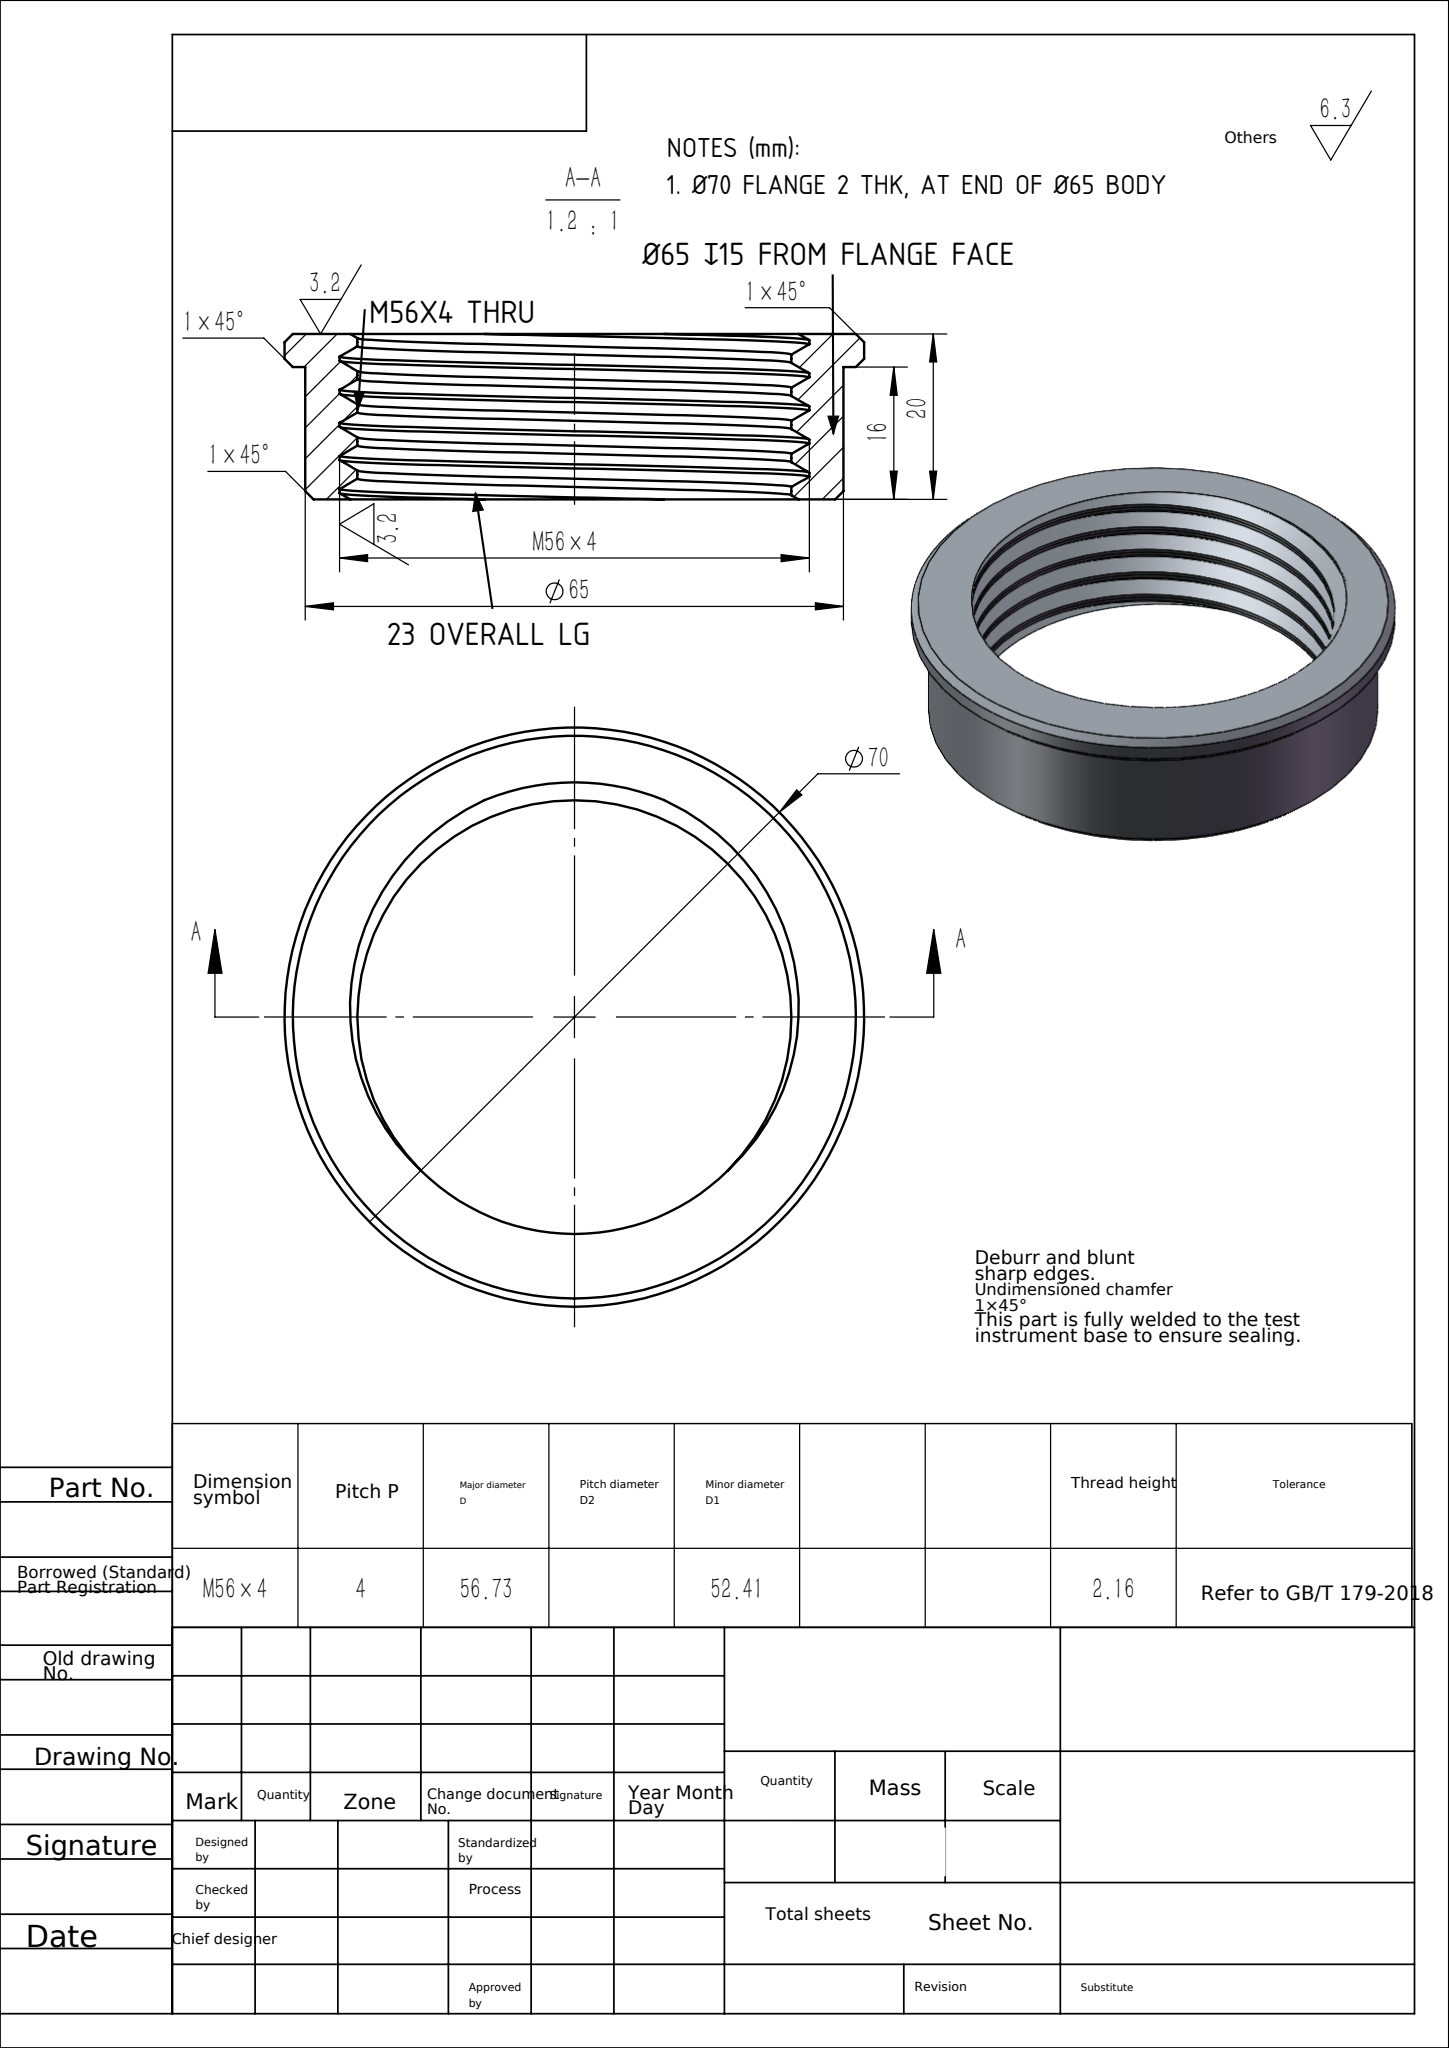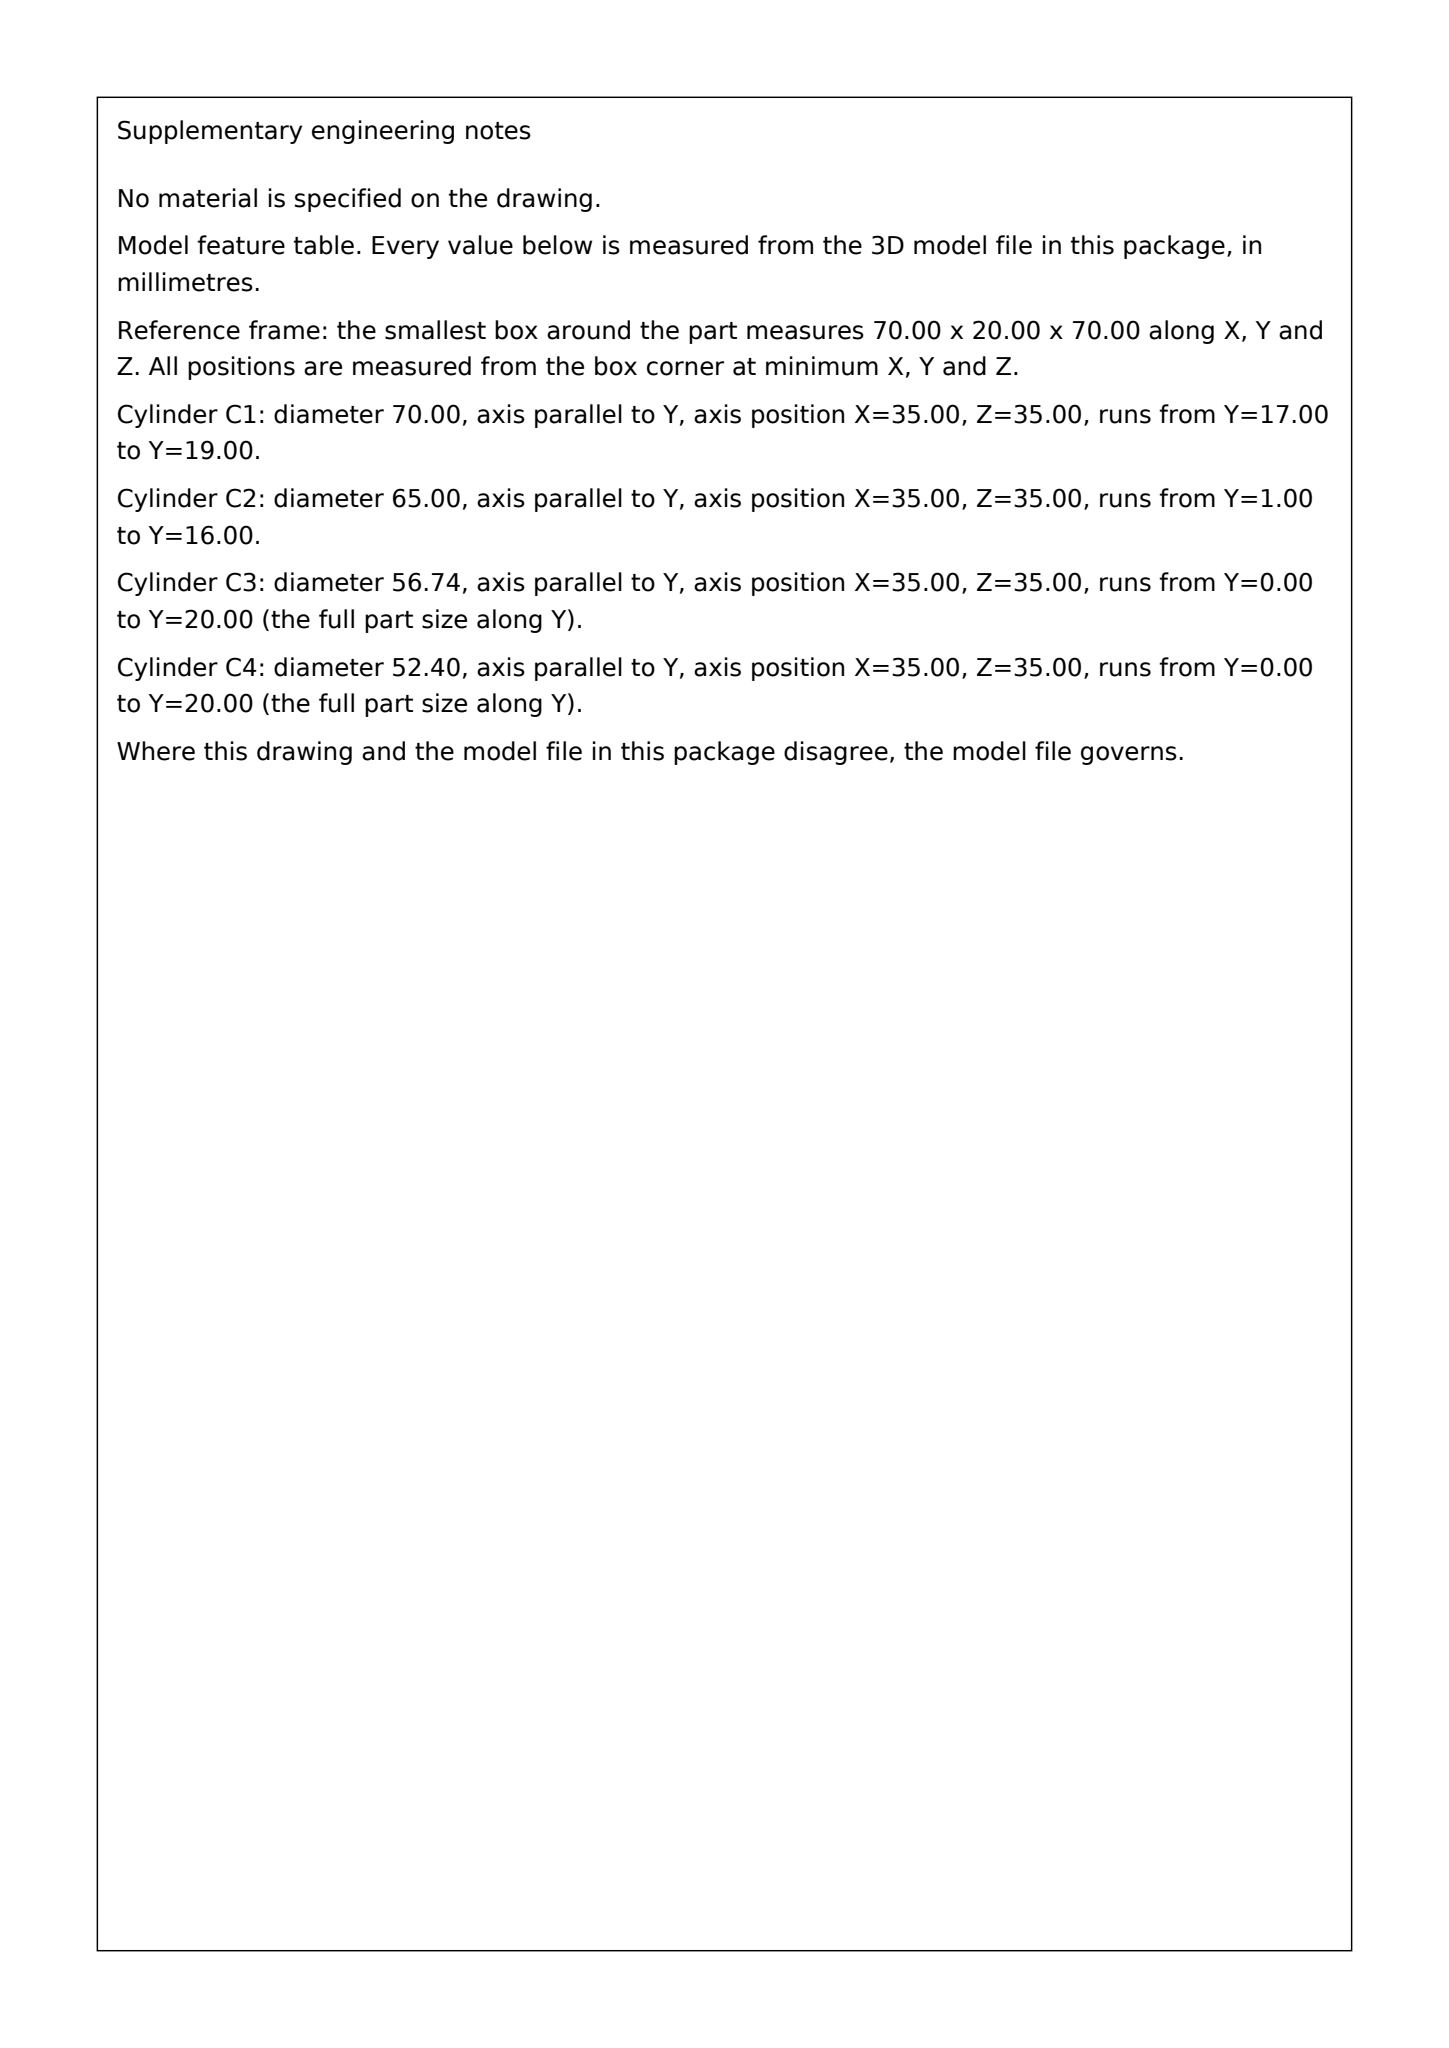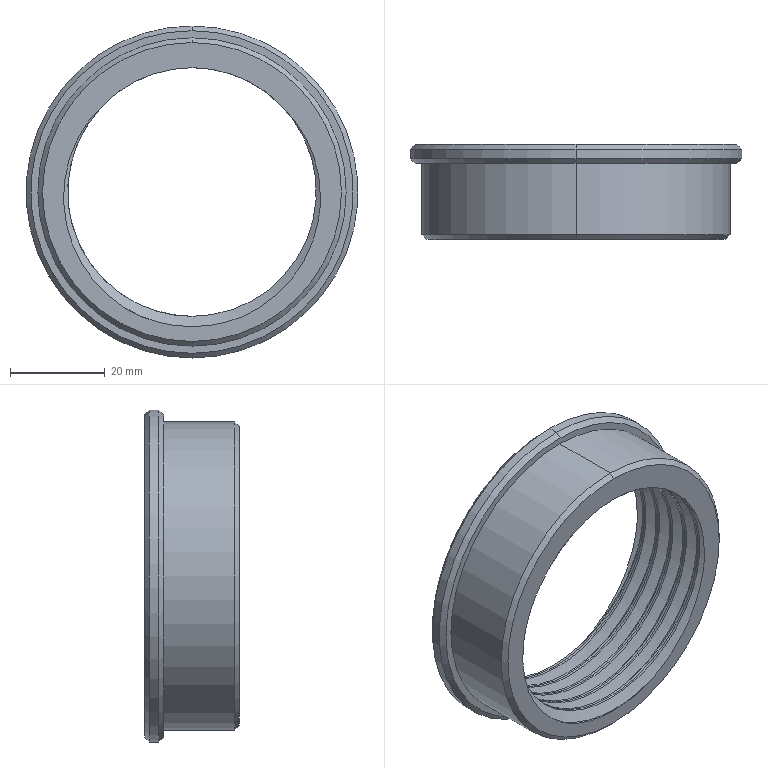Part | SolidWorks | mm | 1 solid | 49 faces | box 70 x 20 x 70 mm | volume 21804 mm3 | cylinder 38 | cone 6 | plane 3 | spline 2 | commonest cylinder face diameters 52.41 x22 56.74 x12 70 x2 65 x2
Drawing notes:
A-A: OVERALL LG 23 | from the solid: bbox_xyz y-extent = 23.001 mm (axis = y)
Ø70 FLANGE 2 THK, AT END OF Ø65 BODY | from the solid: cylinder [dia 70, axis y, length 2.0] adjoining Ø65 cyl
Ø65 OD 15 LG, FROM Ø70 FLANGE FACE | from the solid: cylinder [dia 65, axis y, length 15.0]
THD STARTS AT Ø65 END FACE, RUNS THRU TO Ø70 FLANGE FACE | from the solid: Thread cyls Ø52.41/Ø56.74 span entire 20 between end planes y=1.5 and y=21.5; shoulder plane y=17.5 is flange face